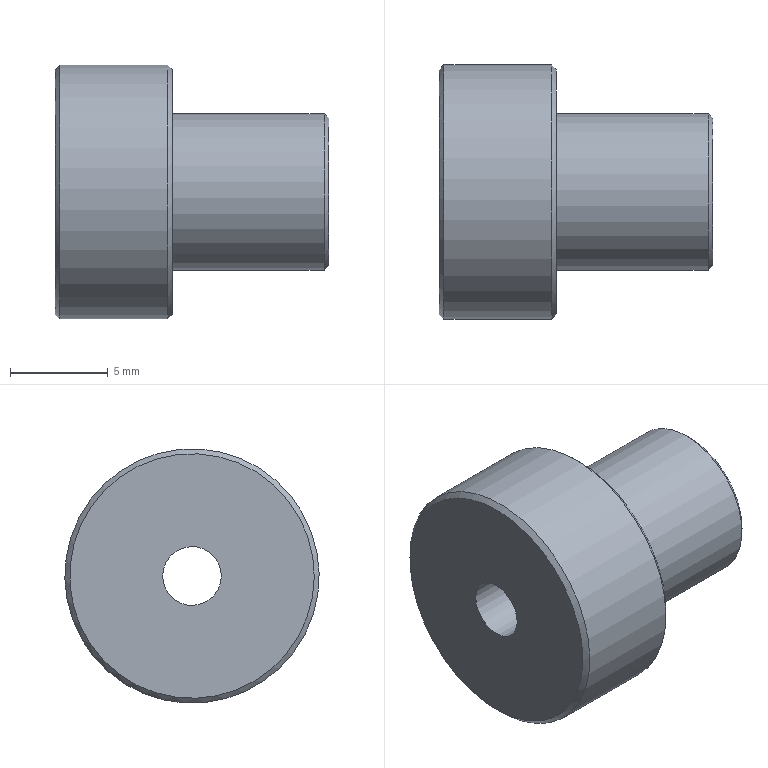Component | NX | PORT_2_2 | 1 solid | 9 faces | box 14 x 13 x 13 mm | volume 1096 mm3 | plane 3 | cylinder 3 | cone 3 | commonest cylinder face diameters 8 x1 13 x1 3 x1
STEP:
#1=CARTESIAN_POINT('',(0.,0.,0.));
#2=DIRECTION('',(0.,0.,1.));
#3=DIRECTION('',(1.,0.,0.));
#4=AXIS2_PLACEMENT_3D('',#1,#2,#3);
#5=CARTESIAN_POINT('',(77.,-10.177,39.614));
#6=VERTEX_POINT('',#5);
#7=CARTESIAN_POINT('',(77.,-11.323,42.386));
#8=VERTEX_POINT('',#7);
#9=CARTESIAN_POINT('',(77.,-10.75,41.));
#10=DIRECTION('',(1.,0.,0.));
#11=DIRECTION('',(0.,0.3818,-0.9242));
#12=AXIS2_PLACEMENT_3D('',#9,#10,#11);
#13=CIRCLE('',#12,1.5);
#14=CARTESIAN_POINT('',(77.,-10.75,41.));
#15=DIRECTION('',(1.,0.,0.));
#16=DIRECTION('',(0.,0.3818,-0.9242));
#17=AXIS2_PLACEMENT_3D('',#14,#15,#16);
#18=PLANE('',#17);
#19=CARTESIAN_POINT('',(0.,0.));
#20=DIRECTION('',(1.,-0.));
#21=AXIS2_PLACEMENT_2D('',#19,#20);
#22=CIRCLE('',#21,1.5);
#23=(GEOMETRIC_REPRESENTATION_CONTEXT(2)PARAMETRIC_REPRESENTATION_CONTEXT()REPRESENTATION_CONTEXT('',''));
#24=DEFINITIONAL_REPRESENTATION('',(#22),#23);
#25=PCURVE('',#18,#24);
#26=CARTESIAN_POINT('',(88.,-10.75,41.));
#27=DIRECTION('',(-1.,0.,0.));
#28=DIRECTION('',(0.,-0.3818,0.9242));
#29=AXIS2_PLACEMENT_3D('',#26,#27,#28);
#30=CYLINDRICAL_SURFACE('',#29,1.5);
#31=CARTESIAN_POINT('',(3.142,11.));
#32=DIRECTION('',(-1.,0.));
#33=VECTOR('',#32,1.);
#34=LINE('',#31,#33);
#35=(GEOMETRIC_REPRESENTATION_CONTEXT(2)PARAMETRIC_REPRESENTATION_CONTEXT()REPRESENTATION_CONTEXT('',''));
#36=DEFINITIONAL_REPRESENTATION('',(#34),#35);
#37=PCURVE('',#30,#36);
#38=SURFACE_CURVE('',#13,(#25,#37),.PCURVE_S1.);
#39=EDGE_CURVE('',#6,#8,#38,.T.);
#40=ORIENTED_EDGE('',*,*,#39,.F.);
#41=CARTESIAN_POINT('',(77.,-10.75,41.));
#42=DIRECTION('',(1.,0.,0.));
#43=DIRECTION('',(0.,0.3818,-0.9242));
#44=AXIS2_PLACEMENT_3D('',#41,#42,#43);
#45=CIRCLE('',#44,1.5);
#46=CARTESIAN_POINT('',(0.,0.));
#47=DIRECTION('',(1.,-0.));
#48=AXIS2_PLACEMENT_2D('',#46,#47);
#49=CIRCLE('',#48,1.5);
#50=(GEOMETRIC_REPRESENTATION_CONTEXT(2)PARAMETRIC_REPRESENTATION_CONTEXT()REPRESENTATION_CONTEXT('',''));
#51=DEFINITIONAL_REPRESENTATION('',(#49),#50);
#52=PCURVE('',#18,#51);
#53=CARTESIAN_POINT('',(9.425,11.));
#54=DIRECTION('',(-1.,0.));
#55=VECTOR('',#54,1.);
#56=LINE('',#53,#55);
#57=(GEOMETRIC_REPRESENTATION_CONTEXT(2)PARAMETRIC_REPRESENTATION_CONTEXT()REPRESENTATION_CONTEXT('',''));
#58=DEFINITIONAL_REPRESENTATION('',(#56),#57);
#59=PCURVE('',#30,#58);
#60=SURFACE_CURVE('',#45,(#52,#59),.PCURVE_S1.);
#61=EDGE_CURVE('',#8,#6,#60,.T.);
#62=ORIENTED_EDGE('',*,*,#61,.F.);
#63=EDGE_LOOP('',(#40,#62));
#64=FACE_BOUND('',#63,.T.);
#65=CARTESIAN_POINT('',(77.,-9.318,37.534));
#66=VERTEX_POINT('',#65);
#67=CARTESIAN_POINT('',(77.,-10.75,41.));
#68=DIRECTION('',(1.,0.,0.));
#69=DIRECTION('',(0.,0.3818,-0.9242));
#70=AXIS2_PLACEMENT_3D('',#67,#68,#69);
#71=CIRCLE('',#70,3.75);
#72=CARTESIAN_POINT('',(0.,0.));
#73=DIRECTION('',(1.,-0.));
#74=AXIS2_PLACEMENT_2D('',#72,#73);
#75=CIRCLE('',#74,3.75);
#76=(GEOMETRIC_REPRESENTATION_CONTEXT(2)PARAMETRIC_REPRESENTATION_CONTEXT()REPRESENTATION_CONTEXT('',''));
#77=DEFINITIONAL_REPRESENTATION('',(#75),#76);
#78=PCURVE('',#18,#77);
#79=CARTESIAN_POINT('',(76.75,-10.75,41.));
#80=DIRECTION('',(-1.,0.,0.));
#81=DIRECTION('',(0.,-0.3818,0.9242));
#82=AXIS2_PLACEMENT_3D('',#79,#80,#81);
#83=CONICAL_SURFACE('',#82,4.,0.7854);
#84=CARTESIAN_POINT('',(9.425,-0.25));
#85=DIRECTION('',(-1.,0.));
#86=VECTOR('',#85,1.);
#87=LINE('',#84,#86);
#88=(GEOMETRIC_REPRESENTATION_CONTEXT(2)PARAMETRIC_REPRESENTATION_CONTEXT()REPRESENTATION_CONTEXT('',''));
#89=DEFINITIONAL_REPRESENTATION('',(#87),#88);
#90=PCURVE('',#83,#89);
#91=SURFACE_CURVE('',#71,(#78,#90),.PCURVE_S1.);
#92=EDGE_CURVE('',#66,#66,#91,.T.);
#93=ORIENTED_EDGE('',*,*,#92,.T.);
#94=EDGE_LOOP('',(#93));
#95=FACE_BOUND('',#94,.T.);
#96=ADVANCED_FACE('',(#64,#95),#18,.T.);
#97=CARTESIAN_POINT('',(76.75,-9.223,37.303));
#98=VERTEX_POINT('',#97);
#99=CARTESIAN_POINT('',(76.75,-12.277,44.697));
#100=VERTEX_POINT('',#99);
#101=CARTESIAN_POINT('',(76.75,-10.75,41.));
#102=DIRECTION('',(-1.,0.,0.));
#103=DIRECTION('',(0.,0.3818,-0.9242));
#104=AXIS2_PLACEMENT_3D('',#101,#102,#103);
#105=CIRCLE('',#104,4.);
#106=CARTESIAN_POINT('',(77.,-10.75,41.));
#107=DIRECTION('',(-1.,0.,0.));
#108=DIRECTION('',(0.,-0.3818,0.9242));
#109=AXIS2_PLACEMENT_3D('',#106,#107,#108);
#110=CYLINDRICAL_SURFACE('',#109,4.);
#111=CARTESIAN_POINT('',(3.142,0.25));
#112=DIRECTION('',(1.,0.));
#113=VECTOR('',#112,1.);
#114=LINE('',#111,#113);
#115=(GEOMETRIC_REPRESENTATION_CONTEXT(2)PARAMETRIC_REPRESENTATION_CONTEXT()REPRESENTATION_CONTEXT('',''));
#116=DEFINITIONAL_REPRESENTATION('',(#114),#115);
#117=PCURVE('',#110,#116);
#118=CARTESIAN_POINT('',(3.142,0.));
#119=DIRECTION('',(1.,0.));
#120=VECTOR('',#119,1.);
#121=LINE('',#118,#120);
#122=(GEOMETRIC_REPRESENTATION_CONTEXT(2)PARAMETRIC_REPRESENTATION_CONTEXT()REPRESENTATION_CONTEXT('',''));
#123=DEFINITIONAL_REPRESENTATION('',(#121),#122);
#124=PCURVE('',#83,#123);
#125=SURFACE_CURVE('',#105,(#117,#124),.PCURVE_S1.);
#126=EDGE_CURVE('',#98,#100,#125,.T.);
#127=ORIENTED_EDGE('',*,*,#126,.T.);
#128=CARTESIAN_POINT('',(69.,-12.277,44.697));
#129=VERTEX_POINT('',#128);
#130=CARTESIAN_POINT('',(76.75,-12.277,44.697));
#131=CARTESIAN_POINT('',(69.,-12.277,44.697));
#132=B_SPLINE_CURVE_WITH_KNOTS('',1,(#130,#131),.UNSPECIFIED.,.F.,.F.,(2,2),(0.25,8.),.PIECEWISE_BEZIER_KNOTS.);
#133=CARTESIAN_POINT('',(6.283,0.));
#134=DIRECTION('',(0.,1.));
#135=VECTOR('',#134,1.);
#136=LINE('',#133,#135);
#137=(GEOMETRIC_REPRESENTATION_CONTEXT(2)PARAMETRIC_REPRESENTATION_CONTEXT()REPRESENTATION_CONTEXT('',''));
#138=DEFINITIONAL_REPRESENTATION('',(#136),#137);
#139=PCURVE('',#110,#138);
#140=CARTESIAN_POINT('',(0.,0.));
#141=DIRECTION('',(0.,1.));
#142=VECTOR('',#141,1.);
#143=LINE('',#140,#142);
#144=(GEOMETRIC_REPRESENTATION_CONTEXT(2)PARAMETRIC_REPRESENTATION_CONTEXT()REPRESENTATION_CONTEXT('',''));
#145=DEFINITIONAL_REPRESENTATION('',(#143),#144);
#146=PCURVE('',#110,#145);
#147=SEAM_CURVE('',#132,(#139,#146),.PCURVE_S1.);
#148=EDGE_CURVE('',#100,#129,#147,.T.);
#149=ORIENTED_EDGE('',*,*,#148,.T.);
#150=CARTESIAN_POINT('',(69.,-10.75,41.));
#151=DIRECTION('',(1.,0.,0.));
#152=DIRECTION('',(0.,-0.3818,0.9242));
#153=AXIS2_PLACEMENT_3D('',#150,#151,#152);
#154=CIRCLE('',#153,4.);
#155=CARTESIAN_POINT('',(6.283,8.));
#156=DIRECTION('',(-1.,0.));
#157=VECTOR('',#156,1.);
#158=LINE('',#155,#157);
#159=(GEOMETRIC_REPRESENTATION_CONTEXT(2)PARAMETRIC_REPRESENTATION_CONTEXT()REPRESENTATION_CONTEXT('',''));
#160=DEFINITIONAL_REPRESENTATION('',(#158),#159);
#161=PCURVE('',#110,#160);
#162=CARTESIAN_POINT('',(69.,-10.75,41.));
#163=DIRECTION('',(1.,0.,0.));
#164=DIRECTION('',(0.,0.3818,-0.9242));
#165=AXIS2_PLACEMENT_3D('',#162,#163,#164);
#166=PLANE('',#165);
#167=CARTESIAN_POINT('',(0.,0.));
#168=DIRECTION('',(-1.,0.));
#169=AXIS2_PLACEMENT_2D('',#167,#168);
#170=CIRCLE('',#169,4.);
#171=(GEOMETRIC_REPRESENTATION_CONTEXT(2)PARAMETRIC_REPRESENTATION_CONTEXT()REPRESENTATION_CONTEXT('',''));
#172=DEFINITIONAL_REPRESENTATION('',(#170),#171);
#173=PCURVE('',#166,#172);
#174=SURFACE_CURVE('',#154,(#161,#173),.PCURVE_S1.);
#175=EDGE_CURVE('',#129,#129,#174,.T.);
#176=ORIENTED_EDGE('',*,*,#175,.T.);
#177=ORIENTED_EDGE('',*,*,#148,.F.);
#178=CARTESIAN_POINT('',(76.75,-10.75,41.));
#179=DIRECTION('',(-1.,0.,0.));
#180=DIRECTION('',(0.,0.3818,-0.9242));
#181=AXIS2_PLACEMENT_3D('',#178,#179,#180);
#182=CIRCLE('',#181,4.);
#183=CARTESIAN_POINT('',(-3.142,0.25));
#184=DIRECTION('',(1.,0.));
#185=VECTOR('',#184,1.);
#186=LINE('',#183,#185);
#187=(GEOMETRIC_REPRESENTATION_CONTEXT(2)PARAMETRIC_REPRESENTATION_CONTEXT()REPRESENTATION_CONTEXT('',''));
#188=DEFINITIONAL_REPRESENTATION('',(#186),#187);
#189=PCURVE('',#110,#188);
#190=CARTESIAN_POINT('',(3.142,0.));
#191=DIRECTION('',(1.,0.));
#192=VECTOR('',#191,1.);
#193=LINE('',#190,#192);
#194=(GEOMETRIC_REPRESENTATION_CONTEXT(2)PARAMETRIC_REPRESENTATION_CONTEXT()REPRESENTATION_CONTEXT('',''));
#195=DEFINITIONAL_REPRESENTATION('',(#193),#194);
#196=PCURVE('',#83,#195);
#197=SURFACE_CURVE('',#182,(#189,#196),.PCURVE_S1.);
#198=EDGE_CURVE('',#100,#98,#197,.T.);
#199=ORIENTED_EDGE('',*,*,#198,.T.);
#200=EDGE_LOOP('',(#127,#149,#176,#177,#199));
#201=FACE_BOUND('',#200,.T.);
#202=ADVANCED_FACE('',(#201),#110,.T.);
#203=CARTESIAN_POINT('',(63.,-11.323,42.386));
#204=VERTEX_POINT('',#203);
#205=CARTESIAN_POINT('',(63.,-10.75,41.));
#206=DIRECTION('',(-1.,0.,0.));
#207=DIRECTION('',(0.,-0.3818,0.9242));
#208=AXIS2_PLACEMENT_3D('',#205,#206,#207);
#209=CIRCLE('',#208,1.5);
#210=CARTESIAN_POINT('',(63.,-10.75,41.));
#211=DIRECTION('',(-1.,0.,0.));
#212=DIRECTION('',(0.,-0.3818,0.9242));
#213=AXIS2_PLACEMENT_3D('',#210,#211,#212);
#214=PLANE('',#213);
#215=CARTESIAN_POINT('',(0.,0.));
#216=DIRECTION('',(1.,0.));
#217=AXIS2_PLACEMENT_2D('',#215,#216);
#218=CIRCLE('',#217,1.5);
#219=(GEOMETRIC_REPRESENTATION_CONTEXT(2)PARAMETRIC_REPRESENTATION_CONTEXT()REPRESENTATION_CONTEXT('',''));
#220=DEFINITIONAL_REPRESENTATION('',(#218),#219);
#221=PCURVE('',#214,#220);
#222=CARTESIAN_POINT('',(0.,25.));
#223=DIRECTION('',(1.,0.));
#224=VECTOR('',#223,1.);
#225=LINE('',#222,#224);
#226=(GEOMETRIC_REPRESENTATION_CONTEXT(2)PARAMETRIC_REPRESENTATION_CONTEXT()REPRESENTATION_CONTEXT('',''));
#227=DEFINITIONAL_REPRESENTATION('',(#225),#226);
#228=PCURVE('',#30,#227);
#229=SURFACE_CURVE('',#209,(#221,#228),.PCURVE_S1.);
#230=EDGE_CURVE('',#204,#204,#229,.T.);
#231=ORIENTED_EDGE('',*,*,#230,.F.);
#232=EDGE_LOOP('',(#231));
#233=FACE_BOUND('',#232,.T.);
#234=CARTESIAN_POINT('',(63.,-13.137,46.776));
#235=VERTEX_POINT('',#234);
#236=CARTESIAN_POINT('',(63.,-10.75,41.));
#237=DIRECTION('',(-1.,0.,0.));
#238=DIRECTION('',(0.,-0.3818,0.9242));
#239=AXIS2_PLACEMENT_3D('',#236,#237,#238);
#240=CIRCLE('',#239,6.25);
#241=CARTESIAN_POINT('',(0.,0.));
#242=DIRECTION('',(1.,0.));
#243=AXIS2_PLACEMENT_2D('',#241,#242);
#244=CIRCLE('',#243,6.25);
#245=(GEOMETRIC_REPRESENTATION_CONTEXT(2)PARAMETRIC_REPRESENTATION_CONTEXT()REPRESENTATION_CONTEXT('',''));
#246=DEFINITIONAL_REPRESENTATION('',(#244),#245);
#247=PCURVE('',#214,#246);
#248=CARTESIAN_POINT('',(63.,-10.75,41.));
#249=DIRECTION('',(1.,0.,0.));
#250=DIRECTION('',(0.,0.3818,-0.9242));
#251=AXIS2_PLACEMENT_3D('',#248,#249,#250);
#252=CONICAL_SURFACE('',#251,6.25,0.7854);
#253=CARTESIAN_POINT('',(9.425,0.));
#254=DIRECTION('',(-1.,0.));
#255=VECTOR('',#254,1.);
#256=LINE('',#253,#255);
#257=(GEOMETRIC_REPRESENTATION_CONTEXT(2)PARAMETRIC_REPRESENTATION_CONTEXT()REPRESENTATION_CONTEXT('',''));
#258=DEFINITIONAL_REPRESENTATION('',(#256),#257);
#259=PCURVE('',#252,#258);
#260=SURFACE_CURVE('',#240,(#247,#259),.PCURVE_S1.);
#261=EDGE_CURVE('',#235,#235,#260,.T.);
#262=ORIENTED_EDGE('',*,*,#261,.T.);
#263=EDGE_LOOP('',(#262));
#264=FACE_BOUND('',#263,.T.);
#265=ADVANCED_FACE('',(#233,#264),#214,.T.);
#266=CARTESIAN_POINT('',(69.,-8.363,35.224));
#267=VERTEX_POINT('',#266);
#268=CARTESIAN_POINT('',(69.,-10.75,41.));
#269=DIRECTION('',(1.,0.,0.));
#270=DIRECTION('',(0.,0.3818,-0.9242));
#271=AXIS2_PLACEMENT_3D('',#268,#269,#270);
#272=CIRCLE('',#271,6.25);
#273=CARTESIAN_POINT('',(0.,0.));
#274=DIRECTION('',(1.,-0.));
#275=AXIS2_PLACEMENT_2D('',#273,#274);
#276=CIRCLE('',#275,6.25);
#277=(GEOMETRIC_REPRESENTATION_CONTEXT(2)PARAMETRIC_REPRESENTATION_CONTEXT()REPRESENTATION_CONTEXT('',''));
#278=DEFINITIONAL_REPRESENTATION('',(#276),#277);
#279=PCURVE('',#166,#278);
#280=CARTESIAN_POINT('',(68.75,-10.75,41.));
#281=DIRECTION('',(-1.,0.,0.));
#282=DIRECTION('',(0.,-0.3818,0.9242));
#283=AXIS2_PLACEMENT_3D('',#280,#281,#282);
#284=CONICAL_SURFACE('',#283,6.5,0.7854);
#285=CARTESIAN_POINT('',(9.425,-0.25));
#286=DIRECTION('',(-1.,0.));
#287=VECTOR('',#286,1.);
#288=LINE('',#285,#287);
#289=(GEOMETRIC_REPRESENTATION_CONTEXT(2)PARAMETRIC_REPRESENTATION_CONTEXT()REPRESENTATION_CONTEXT('',''));
#290=DEFINITIONAL_REPRESENTATION('',(#288),#289);
#291=PCURVE('',#284,#290);
#292=SURFACE_CURVE('',#272,(#279,#291),.PCURVE_S1.);
#293=EDGE_CURVE('',#267,#267,#292,.T.);
#294=ORIENTED_EDGE('',*,*,#293,.T.);
#295=EDGE_LOOP('',(#294));
#296=FACE_BOUND('',#295,.T.);
#297=ORIENTED_EDGE('',*,*,#175,.F.);
#298=EDGE_LOOP('',(#297));
#299=FACE_BOUND('',#298,.T.);
#300=ADVANCED_FACE('',(#296,#299),#166,.T.);
#301=CARTESIAN_POINT('',(63.25,-13.232,47.007));
#302=VERTEX_POINT('',#301);
#303=CARTESIAN_POINT('',(63.25,-10.75,41.));
#304=DIRECTION('',(1.,0.,0.));
#305=DIRECTION('',(0.,-0.3818,0.9242));
#306=AXIS2_PLACEMENT_3D('',#303,#304,#305);
#307=CIRCLE('',#306,6.5);
#308=CARTESIAN_POINT('',(69.,-10.75,41.));
#309=DIRECTION('',(-1.,0.,0.));
#310=DIRECTION('',(0.,-0.3818,0.9242));
#311=AXIS2_PLACEMENT_3D('',#308,#309,#310);
#312=CYLINDRICAL_SURFACE('',#311,6.5);
#313=CARTESIAN_POINT('',(6.283,5.75));
#314=DIRECTION('',(-1.,0.));
#315=VECTOR('',#314,1.);
#316=LINE('',#313,#315);
#317=(GEOMETRIC_REPRESENTATION_CONTEXT(2)PARAMETRIC_REPRESENTATION_CONTEXT()REPRESENTATION_CONTEXT('',''));
#318=DEFINITIONAL_REPRESENTATION('',(#316),#317);
#319=PCURVE('',#312,#318);
#320=CARTESIAN_POINT('',(3.142,0.25));
#321=DIRECTION('',(1.,0.));
#322=VECTOR('',#321,1.);
#323=LINE('',#320,#322);
#324=(GEOMETRIC_REPRESENTATION_CONTEXT(2)PARAMETRIC_REPRESENTATION_CONTEXT()REPRESENTATION_CONTEXT('',''));
#325=DEFINITIONAL_REPRESENTATION('',(#323),#324);
#326=PCURVE('',#252,#325);
#327=SURFACE_CURVE('',#307,(#319,#326),.PCURVE_S1.);
#328=EDGE_CURVE('',#302,#302,#327,.T.);
#329=ORIENTED_EDGE('',*,*,#328,.T.);
#330=CARTESIAN_POINT('',(68.75,-13.232,47.007));
#331=VERTEX_POINT('',#330);
#332=CARTESIAN_POINT('',(68.75,-13.232,47.007));
#333=CARTESIAN_POINT('',(63.25,-13.232,47.007));
#334=B_SPLINE_CURVE_WITH_KNOTS('',1,(#332,#333),.UNSPECIFIED.,.F.,.F.,(2,2),(0.25,5.75),.PIECEWISE_BEZIER_KNOTS.);
#335=CARTESIAN_POINT('',(0.,0.));
#336=DIRECTION('',(0.,1.));
#337=VECTOR('',#336,1.);
#338=LINE('',#335,#337);
#339=(GEOMETRIC_REPRESENTATION_CONTEXT(2)PARAMETRIC_REPRESENTATION_CONTEXT()REPRESENTATION_CONTEXT('',''));
#340=DEFINITIONAL_REPRESENTATION('',(#338),#339);
#341=PCURVE('',#312,#340);
#342=CARTESIAN_POINT('',(6.283,0.));
#343=DIRECTION('',(0.,1.));
#344=VECTOR('',#343,1.);
#345=LINE('',#342,#344);
#346=(GEOMETRIC_REPRESENTATION_CONTEXT(2)PARAMETRIC_REPRESENTATION_CONTEXT()REPRESENTATION_CONTEXT('',''));
#347=DEFINITIONAL_REPRESENTATION('',(#345),#346);
#348=PCURVE('',#312,#347);
#349=SEAM_CURVE('',#334,(#341,#348),.PCURVE_S1.);
#350=EDGE_CURVE('',#331,#302,#349,.T.);
#351=ORIENTED_EDGE('',*,*,#350,.F.);
#352=CARTESIAN_POINT('',(68.75,-8.268,34.993));
#353=VERTEX_POINT('',#352);
#354=CARTESIAN_POINT('',(68.75,-10.75,41.));
#355=DIRECTION('',(-1.,0.,0.));
#356=DIRECTION('',(0.,0.3818,-0.9242));
#357=AXIS2_PLACEMENT_3D('',#354,#355,#356);
#358=CIRCLE('',#357,6.5);
#359=CARTESIAN_POINT('',(-3.142,0.25));
#360=DIRECTION('',(1.,0.));
#361=VECTOR('',#360,1.);
#362=LINE('',#359,#361);
#363=(GEOMETRIC_REPRESENTATION_CONTEXT(2)PARAMETRIC_REPRESENTATION_CONTEXT()REPRESENTATION_CONTEXT('',''));
#364=DEFINITIONAL_REPRESENTATION('',(#362),#363);
#365=PCURVE('',#312,#364);
#366=CARTESIAN_POINT('',(3.142,0.));
#367=DIRECTION('',(1.,-0.));
#368=VECTOR('',#367,1.);
#369=LINE('',#366,#368);
#370=(GEOMETRIC_REPRESENTATION_CONTEXT(2)PARAMETRIC_REPRESENTATION_CONTEXT()REPRESENTATION_CONTEXT('',''));
#371=DEFINITIONAL_REPRESENTATION('',(#369),#370);
#372=PCURVE('',#284,#371);
#373=SURFACE_CURVE('',#358,(#365,#372),.PCURVE_S1.);
#374=EDGE_CURVE('',#331,#353,#373,.T.);
#375=ORIENTED_EDGE('',*,*,#374,.T.);
#376=CARTESIAN_POINT('',(68.75,-10.75,41.));
#377=DIRECTION('',(-1.,0.,0.));
#378=DIRECTION('',(0.,0.3818,-0.9242));
#379=AXIS2_PLACEMENT_3D('',#376,#377,#378);
#380=CIRCLE('',#379,6.5);
#381=CARTESIAN_POINT('',(3.142,0.25));
#382=DIRECTION('',(1.,0.));
#383=VECTOR('',#382,1.);
#384=LINE('',#381,#383);
#385=(GEOMETRIC_REPRESENTATION_CONTEXT(2)PARAMETRIC_REPRESENTATION_CONTEXT()REPRESENTATION_CONTEXT('',''));
#386=DEFINITIONAL_REPRESENTATION('',(#384),#385);
#387=PCURVE('',#312,#386);
#388=CARTESIAN_POINT('',(3.142,0.));
#389=DIRECTION('',(1.,0.));
#390=VECTOR('',#389,1.);
#391=LINE('',#388,#390);
#392=(GEOMETRIC_REPRESENTATION_CONTEXT(2)PARAMETRIC_REPRESENTATION_CONTEXT()REPRESENTATION_CONTEXT('',''));
#393=DEFINITIONAL_REPRESENTATION('',(#391),#392);
#394=PCURVE('',#284,#393);
#395=SURFACE_CURVE('',#380,(#387,#394),.PCURVE_S1.);
#396=EDGE_CURVE('',#353,#331,#395,.T.);
#397=ORIENTED_EDGE('',*,*,#396,.T.);
#398=ORIENTED_EDGE('',*,*,#350,.T.);
#399=EDGE_LOOP('',(#329,#351,#375,#397,#398));
#400=FACE_BOUND('',#399,.T.);
#401=ADVANCED_FACE('',(#400),#312,.T.);
#402=ORIENTED_EDGE('',*,*,#92,.F.);
#403=CARTESIAN_POINT('',(77.,-9.318,37.534));
#404=CARTESIAN_POINT('',(76.75,-9.223,37.303));
#405=B_SPLINE_CURVE_WITH_KNOTS('',1,(#403,#404),.UNSPECIFIED.,.F.,.F.,(2,2),(-0.3536,0.),.PIECEWISE_BEZIER_KNOTS.);
#406=CARTESIAN_POINT('',(9.425,0.));
#407=DIRECTION('',(0.,1.));
#408=VECTOR('',#407,1.);
#409=LINE('',#406,#408);
#410=(GEOMETRIC_REPRESENTATION_CONTEXT(2)PARAMETRIC_REPRESENTATION_CONTEXT()REPRESENTATION_CONTEXT('',''));
#411=DEFINITIONAL_REPRESENTATION('',(#409),#410);
#412=PCURVE('',#83,#411);
#413=CARTESIAN_POINT('',(3.142,0.));
#414=DIRECTION('',(0.,1.));
#415=VECTOR('',#414,1.);
#416=LINE('',#413,#415);
#417=(GEOMETRIC_REPRESENTATION_CONTEXT(2)PARAMETRIC_REPRESENTATION_CONTEXT()REPRESENTATION_CONTEXT('',''));
#418=DEFINITIONAL_REPRESENTATION('',(#416),#417);
#419=PCURVE('',#83,#418);
#420=SEAM_CURVE('',#405,(#412,#419),.PCURVE_S1.);
#421=EDGE_CURVE('',#66,#98,#420,.T.);
#422=ORIENTED_EDGE('',*,*,#421,.T.);
#423=ORIENTED_EDGE('',*,*,#198,.F.);
#424=ORIENTED_EDGE('',*,*,#126,.F.);
#425=ORIENTED_EDGE('',*,*,#421,.F.);
#426=EDGE_LOOP('',(#402,#422,#423,#424,#425));
#427=FACE_BOUND('',#426,.T.);
#428=ADVANCED_FACE('',(#427),#83,.T.);
#429=ORIENTED_EDGE('',*,*,#328,.F.);
#430=CARTESIAN_POINT('',(63.,-13.137,46.776));
#431=CARTESIAN_POINT('',(63.25,-13.232,47.007));
#432=B_SPLINE_CURVE_WITH_KNOTS('',1,(#430,#431),.UNSPECIFIED.,.F.,.F.,(2,2),(0.,0.3536),.PIECEWISE_BEZIER_KNOTS.);
#433=CARTESIAN_POINT('',(3.142,0.));
#434=DIRECTION('',(0.,1.));
#435=VECTOR('',#434,1.);
#436=LINE('',#433,#435);
#437=(GEOMETRIC_REPRESENTATION_CONTEXT(2)PARAMETRIC_REPRESENTATION_CONTEXT()REPRESENTATION_CONTEXT('',''));
#438=DEFINITIONAL_REPRESENTATION('',(#436),#437);
#439=PCURVE('',#252,#438);
#440=CARTESIAN_POINT('',(9.425,0.));
#441=DIRECTION('',(0.,1.));
#442=VECTOR('',#441,1.);
#443=LINE('',#440,#442);
#444=(GEOMETRIC_REPRESENTATION_CONTEXT(2)PARAMETRIC_REPRESENTATION_CONTEXT()REPRESENTATION_CONTEXT('',''));
#445=DEFINITIONAL_REPRESENTATION('',(#443),#444);
#446=PCURVE('',#252,#445);
#447=SEAM_CURVE('',#432,(#439,#446),.PCURVE_S1.);
#448=EDGE_CURVE('',#235,#302,#447,.T.);
#449=ORIENTED_EDGE('',*,*,#448,.F.);
#450=ORIENTED_EDGE('',*,*,#261,.F.);
#451=ORIENTED_EDGE('',*,*,#448,.T.);
#452=EDGE_LOOP('',(#429,#449,#450,#451));
#453=FACE_BOUND('',#452,.T.);
#454=ADVANCED_FACE('',(#453),#252,.T.);
#455=ORIENTED_EDGE('',*,*,#293,.F.);
#456=CARTESIAN_POINT('',(69.,-8.363,35.224));
#457=CARTESIAN_POINT('',(68.75,-8.268,34.993));
#458=B_SPLINE_CURVE_WITH_KNOTS('',1,(#456,#457),.UNSPECIFIED.,.F.,.F.,(2,2),(-0.3536,0.),.PIECEWISE_BEZIER_KNOTS.);
#459=CARTESIAN_POINT('',(9.425,0.));
#460=DIRECTION('',(0.,1.));
#461=VECTOR('',#460,1.);
#462=LINE('',#459,#461);
#463=(GEOMETRIC_REPRESENTATION_CONTEXT(2)PARAMETRIC_REPRESENTATION_CONTEXT()REPRESENTATION_CONTEXT('',''));
#464=DEFINITIONAL_REPRESENTATION('',(#462),#463);
#465=PCURVE('',#284,#464);
#466=CARTESIAN_POINT('',(3.142,0.));
#467=DIRECTION('',(0.,1.));
#468=VECTOR('',#467,1.);
#469=LINE('',#466,#468);
#470=(GEOMETRIC_REPRESENTATION_CONTEXT(2)PARAMETRIC_REPRESENTATION_CONTEXT()REPRESENTATION_CONTEXT('',''));
#471=DEFINITIONAL_REPRESENTATION('',(#469),#470);
#472=PCURVE('',#284,#471);
#473=SEAM_CURVE('',#458,(#465,#472),.PCURVE_S1.);
#474=EDGE_CURVE('',#267,#353,#473,.T.);
#475=ORIENTED_EDGE('',*,*,#474,.T.);
#476=ORIENTED_EDGE('',*,*,#374,.F.);
#477=ORIENTED_EDGE('',*,*,#396,.F.);
#478=ORIENTED_EDGE('',*,*,#474,.F.);
#479=EDGE_LOOP('',(#455,#475,#476,#477,#478));
#480=FACE_BOUND('',#479,.T.);
#481=ADVANCED_FACE('',(#480),#284,.T.);
#482=ORIENTED_EDGE('',*,*,#61,.F.);
#483=CARTESIAN_POINT('',(77.,-11.323,42.386));
#484=CARTESIAN_POINT('',(63.,-11.323,42.386));
#485=B_SPLINE_CURVE_WITH_KNOTS('',1,(#483,#484),.UNSPECIFIED.,.F.,.F.,(2,2),(11.,25.),.PIECEWISE_BEZIER_KNOTS.);
#486=CARTESIAN_POINT('',(6.283,0.));
#487=DIRECTION('',(0.,1.));
#488=VECTOR('',#487,1.);
#489=LINE('',#486,#488);
#490=(GEOMETRIC_REPRESENTATION_CONTEXT(2)PARAMETRIC_REPRESENTATION_CONTEXT()REPRESENTATION_CONTEXT('',''));
#491=DEFINITIONAL_REPRESENTATION('',(#489),#490);
#492=PCURVE('',#30,#491);
#493=CARTESIAN_POINT('',(0.,0.));
#494=DIRECTION('',(0.,1.));
#495=VECTOR('',#494,1.);
#496=LINE('',#493,#495);
#497=(GEOMETRIC_REPRESENTATION_CONTEXT(2)PARAMETRIC_REPRESENTATION_CONTEXT()REPRESENTATION_CONTEXT('',''));
#498=DEFINITIONAL_REPRESENTATION('',(#496),#497);
#499=PCURVE('',#30,#498);
#500=SEAM_CURVE('',#485,(#492,#499),.PCURVE_S1.);
#501=EDGE_CURVE('',#8,#204,#500,.T.);
#502=ORIENTED_EDGE('',*,*,#501,.T.);
#503=ORIENTED_EDGE('',*,*,#230,.F.);
#504=ORIENTED_EDGE('',*,*,#501,.F.);
#505=ORIENTED_EDGE('',*,*,#39,.F.);
#506=EDGE_LOOP('',(#482,#502,#503,#504,#505));
#507=FACE_BOUND('',#506,.F.);
#508=ADVANCED_FACE('',(#507),#30,.F.);
#509=CLOSED_SHELL('',(#96,#202,#265,#300,#401,#428,#454,#481,#508));
#510=MANIFOLD_SOLID_BREP('',#509);
#511=(LENGTH_UNIT()NAMED_UNIT(*)SI_UNIT(.MILLI.,.METRE.));
#512=UNCERTAINTY_MEASURE_WITH_UNIT(LENGTH_MEASURE(0.00001),#511,'','');
#513=(NAMED_UNIT(*)PLANE_ANGLE_UNIT()SI_UNIT($,.RADIAN.));
#514=(NAMED_UNIT(*)SI_UNIT($,.STERADIAN.)SOLID_ANGLE_UNIT());
#515=(GEOMETRIC_REPRESENTATION_CONTEXT(3)GLOBAL_UNCERTAINTY_ASSIGNED_CONTEXT((#512))GLOBAL_UNIT_ASSIGNED_CONTEXT((#511,#513,#514))REPRESENTATION_CONTEXT('',''));
#516=ADVANCED_BREP_SHAPE_REPRESENTATION('',(#4,#510),#515);